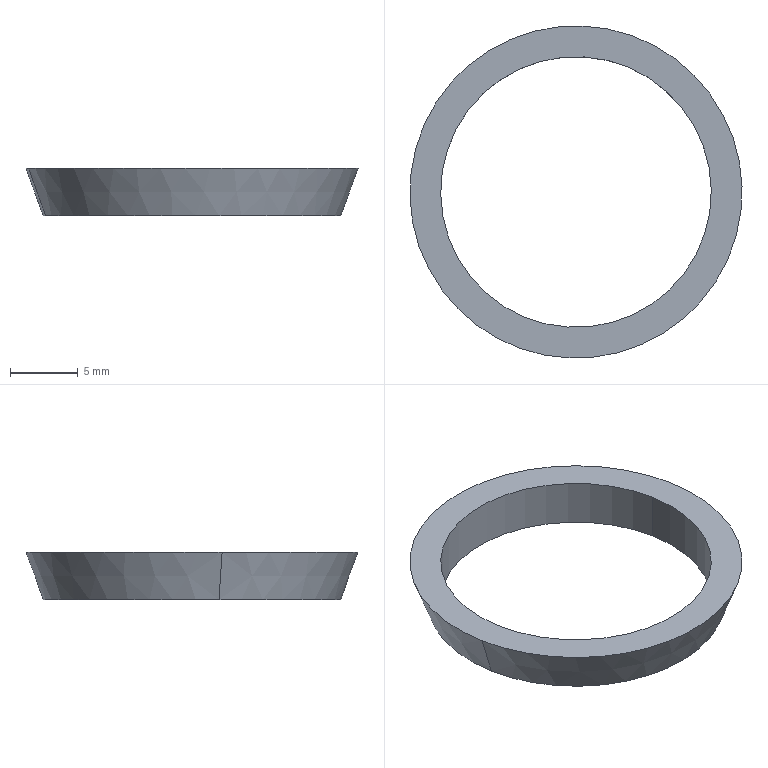Component | SolidWorks | OilSeal-1 | 1 solid | 6 faces | box 24.55 x 24.55 x 3.5 mm | volume 391 mm3 | cylinder 2 | cone 2 | plane 2 | commonest cylinder face diameters 20 x2
build123d program:
from build123d import *

# Parameters (mm, degrees)
SKETCH2_R           = 11
SKETCH2_R_2         = 10
BOSS_EXTRUDE1_DEPTH = 3.5
BOSS_EXTRUDE1_DRAFT = -20
SKETCH3_R           = 10
CUT_EXTRUDE1_DEPTH  = 15.5


with BuildPart() as part:
    # Sketch2 → Boss-Extrude1 (with draft: the straight prism first)
    with BuildSketch(Plane.XY):
        with Locations((-80.719, -28.485)):
            Circle(SKETCH2_R)
        with Locations((-80.719, -28.485)):
            Circle(SKETCH2_R_2, mode=Mode.SUBTRACT)
    extrude(amount=BOSS_EXTRUDE1_DEPTH)
    # Boss-Extrude1: the draft: its side faces are tilted about the plane it starts from
    boss_extrude1_sides = [part.faces().sort_by_distance(p)[0] for p in [
        (-91.719, -28.485, 1.75),
        (-90.719, -28.485, 1.75),
    ]]
    draft(boss_extrude1_sides, Plane.XY, BOSS_EXTRUDE1_DRAFT)

    # Sketch3 → Cut-Extrude1 (cut)
    with BuildSketch(Plane.XY.offset(3.5)):
        with Locations((-80.719, -28.485)):
            Circle(SKETCH3_R)
    extrude(amount=-CUT_EXTRUDE1_DEPTH, mode=Mode.SUBTRACT)


solid = part.part

# Placed as in the assembly
solid = solid.moved(Location((0, 0, 213.536), (0, 0, 0)))
STEP:
#1=COLOUR_RGB('',0.7922,0.8196,0.9333);
#2=FILL_AREA_STYLE_COLOUR('',#1);
#3=FILL_AREA_STYLE('',(#2));
#4=SURFACE_STYLE_FILL_AREA(#3);
#5=SURFACE_SIDE_STYLE('',(#4));
#6=SURFACE_STYLE_USAGE(.BOTH.,#5);
#7=PRESENTATION_STYLE_ASSIGNMENT((#6));
#8=CARTESIAN_POINT('',(-2.791,-1.05,8.407));
#9=VERTEX_POINT('',#8);
#10=CARTESIAN_POINT('',(-3.565,-1.193,8.407));
#11=VERTEX_POINT('',#10);
#12=CARTESIAN_POINT('',(-3.178,-1.121,8.407));
#13=DIRECTION('',(0.,0.,-1.));
#14=DIRECTION('',(-0.9835,-0.1812,0.));
#15=AXIS2_PLACEMENT_3D('',#12,#13,#14);
#16=CIRCLE('',#15,0.3937);
#17=EDGE_CURVE('',#9,#11,#16,.T.);
#18=ORIENTED_EDGE('',*,*,#17,.T.);
#19=CARTESIAN_POINT('',(-3.565,-1.193,8.545));
#20=VERTEX_POINT('',#19);
#21=CARTESIAN_POINT('',(-3.565,-1.193,7.934));
#22=DIRECTION('',(0.,0.,1.));
#23=VECTOR('',#22,39.37);
#24=LINE('',#21,#23);
#25=EDGE_CURVE('',#11,#20,#24,.T.);
#26=ORIENTED_EDGE('',*,*,#25,.T.);
#27=CARTESIAN_POINT('',(-2.791,-1.05,8.545));
#28=VERTEX_POINT('',#27);
#29=CARTESIAN_POINT('',(-3.178,-1.121,8.545));
#30=DIRECTION('',(0.,0.,1.));
#31=DIRECTION('',(0.9835,0.1812,0.));
#32=AXIS2_PLACEMENT_3D('',#29,#30,#31);
#33=CIRCLE('',#32,0.3937);
#34=EDGE_CURVE('',#20,#28,#33,.T.);
#35=ORIENTED_EDGE('',*,*,#34,.T.);
#36=CARTESIAN_POINT('',(-2.791,-1.05,7.934));
#37=DIRECTION('',(0.,0.,1.));
#38=VECTOR('',#37,39.37);
#39=LINE('',#36,#38);
#40=EDGE_CURVE('',#9,#28,#39,.T.);
#41=ORIENTED_EDGE('',*,*,#40,.F.);
#42=EDGE_LOOP('',(#18,#26,#35,#41));
#43=FACE_OUTER_BOUND('',#42,.T.);
#44=CARTESIAN_POINT('',(-3.178,-1.121,7.934));
#45=DIRECTION('',(0.,0.,1.));
#46=DIRECTION('',(0.9835,0.1812,0.));
#47=AXIS2_PLACEMENT_3D('',#44,#45,#46);
#48=CYLINDRICAL_SURFACE('',#47,0.3937);
#49=ADVANCED_FACE('',(#43),#48,.F.);
#50=CARTESIAN_POINT('',(-2.752,-1.043,8.407));
#51=VERTEX_POINT('',#50);
#52=CARTESIAN_POINT('',(-3.604,-1.2,8.407));
#53=VERTEX_POINT('',#52);
#54=CARTESIAN_POINT('',(-3.178,-1.121,8.407));
#55=DIRECTION('',(0.,0.,1.));
#56=DIRECTION('',(0.9835,0.1812,0.));
#57=AXIS2_PLACEMENT_3D('',#54,#55,#56);
#58=CIRCLE('',#57,0.4331);
#59=EDGE_CURVE('',#51,#53,#58,.T.);
#60=ORIENTED_EDGE('',*,*,#59,.T.);
#61=CARTESIAN_POINT('',(-3.653,-1.209,8.545));
#62=VERTEX_POINT('',#61);
#63=CARTESIAN_POINT('',(-3.604,-1.2,8.407));
#64=DIRECTION('',(-0.3364,-0.06196,0.9397));
#65=VECTOR('',#64,39.37);
#66=LINE('',#63,#65);
#67=EDGE_CURVE('',#53,#62,#66,.T.);
#68=ORIENTED_EDGE('',*,*,#67,.T.);
#69=CARTESIAN_POINT('',(-2.703,-1.034,8.545));
#70=VERTEX_POINT('',#69);
#71=CARTESIAN_POINT('',(-3.178,-1.121,8.545));
#72=DIRECTION('',(0.,0.,1.));
#73=DIRECTION('',(0.9835,0.1812,0.));
#74=AXIS2_PLACEMENT_3D('',#71,#72,#73);
#75=CIRCLE('',#74,0.4832);
#76=EDGE_CURVE('',#70,#62,#75,.T.);
#77=ORIENTED_EDGE('',*,*,#76,.F.);
#78=CARTESIAN_POINT('',(-2.752,-1.043,8.407));
#79=DIRECTION('',(0.3364,0.06196,0.9397));
#80=VECTOR('',#79,39.37);
#81=LINE('',#78,#80);
#82=EDGE_CURVE('',#51,#70,#81,.T.);
#83=ORIENTED_EDGE('',*,*,#82,.F.);
#84=EDGE_LOOP('',(#60,#68,#77,#83));
#85=FACE_OUTER_BOUND('',#84,.T.);
#86=CARTESIAN_POINT('',(-3.178,-1.121,8.407));
#87=DIRECTION('',(0.,0.,1.));
#88=DIRECTION('',(0.9835,0.1812,0.));
#89=AXIS2_PLACEMENT_3D('',#86,#87,#88);
#90=CONICAL_SURFACE('',#89,0.4331,0.3491);
#91=ADVANCED_FACE('',(#85),#90,.T.);
#92=CARTESIAN_POINT('',(-3.178,-1.121,8.545));
#93=DIRECTION('',(0.,0.,1.));
#94=DIRECTION('',(0.9835,0.1812,0.));
#95=AXIS2_PLACEMENT_3D('',#92,#93,#94);
#96=CIRCLE('',#95,0.3937);
#97=EDGE_CURVE('',#28,#20,#96,.T.);
#98=ORIENTED_EDGE('',*,*,#97,.F.);
#99=ORIENTED_EDGE('',*,*,#34,.F.);
#100=EDGE_LOOP('',(#98,#99));
#101=FACE_BOUND('',#100,.T.);
#102=ORIENTED_EDGE('',*,*,#76,.T.);
#103=CARTESIAN_POINT('',(-3.178,-1.121,8.545));
#104=DIRECTION('',(0.,0.,1.));
#105=DIRECTION('',(0.9835,0.1812,0.));
#106=AXIS2_PLACEMENT_3D('',#103,#104,#105);
#107=CIRCLE('',#106,0.4832);
#108=EDGE_CURVE('',#62,#70,#107,.T.);
#109=ORIENTED_EDGE('',*,*,#108,.T.);
#110=EDGE_LOOP('',(#102,#109));
#111=FACE_OUTER_BOUND('',#110,.T.);
#112=CARTESIAN_POINT('',(-3.178,-1.121,8.545));
#113=DIRECTION('',(0.,0.,1.));
#114=DIRECTION('',(0.9835,0.1812,0.));
#115=AXIS2_PLACEMENT_3D('',#112,#113,#114);
#116=PLANE('',#115);
#117=ADVANCED_FACE('',(#101,#111),#116,.T.);
#118=ORIENTED_EDGE('',*,*,#59,.F.);
#119=CARTESIAN_POINT('',(-3.178,-1.121,8.407));
#120=DIRECTION('',(0.,0.,1.));
#121=DIRECTION('',(0.9835,0.1812,0.));
#122=AXIS2_PLACEMENT_3D('',#119,#120,#121);
#123=CIRCLE('',#122,0.4331);
#124=EDGE_CURVE('',#53,#51,#123,.T.);
#125=ORIENTED_EDGE('',*,*,#124,.F.);
#126=EDGE_LOOP('',(#118,#125));
#127=FACE_OUTER_BOUND('',#126,.T.);
#128=ORIENTED_EDGE('',*,*,#17,.F.);
#129=CARTESIAN_POINT('',(-3.178,-1.121,8.407));
#130=DIRECTION('',(0.,0.,-1.));
#131=DIRECTION('',(-0.9835,-0.1812,0.));
#132=AXIS2_PLACEMENT_3D('',#129,#130,#131);
#133=CIRCLE('',#132,0.3937);
#134=EDGE_CURVE('',#11,#9,#133,.T.);
#135=ORIENTED_EDGE('',*,*,#134,.F.);
#136=EDGE_LOOP('',(#128,#135));
#137=FACE_BOUND('',#136,.T.);
#138=CARTESIAN_POINT('',(-3.178,-1.121,8.407));
#139=DIRECTION('',(0.,0.,1.));
#140=DIRECTION('',(0.9835,0.1812,0.));
#141=AXIS2_PLACEMENT_3D('',#138,#139,#140);
#142=PLANE('',#141);
#143=ADVANCED_FACE('',(#127,#137),#142,.F.);
#144=ORIENTED_EDGE('',*,*,#67,.F.);
#145=ORIENTED_EDGE('',*,*,#124,.T.);
#146=ORIENTED_EDGE('',*,*,#82,.T.);
#147=ORIENTED_EDGE('',*,*,#108,.F.);
#148=EDGE_LOOP('',(#144,#145,#146,#147));
#149=FACE_OUTER_BOUND('',#148,.T.);
#150=CARTESIAN_POINT('',(-3.178,-1.121,8.407));
#151=DIRECTION('',(0.,0.,1.));
#152=DIRECTION('',(0.9835,0.1812,0.));
#153=AXIS2_PLACEMENT_3D('',#150,#151,#152);
#154=CONICAL_SURFACE('',#153,0.4331,0.3491);
#155=ADVANCED_FACE('',(#149),#154,.T.);
#156=ORIENTED_EDGE('',*,*,#25,.F.);
#157=ORIENTED_EDGE('',*,*,#134,.T.);
#158=ORIENTED_EDGE('',*,*,#40,.T.);
#159=ORIENTED_EDGE('',*,*,#97,.T.);
#160=EDGE_LOOP('',(#156,#157,#158,#159));
#161=FACE_OUTER_BOUND('',#160,.T.);
#162=CARTESIAN_POINT('',(-3.178,-1.121,7.934));
#163=DIRECTION('',(0.,0.,1.));
#164=DIRECTION('',(0.9835,0.1812,0.));
#165=AXIS2_PLACEMENT_3D('',#162,#163,#164);
#166=CYLINDRICAL_SURFACE('',#165,0.3937);
#167=ADVANCED_FACE('',(#161),#166,.F.);
#168=CLOSED_SHELL('',(#49,#91,#117,#143,#155,#167));
#169=MANIFOLD_SOLID_BREP('',#168);
#170=STYLED_ITEM('',(#7),#169);
#171=(LENGTH_UNIT()NAMED_UNIT(*)SI_UNIT($,.METRE.));
#172=LENGTH_MEASURE_WITH_UNIT(LENGTH_MEASURE(0.0254),#171);
#173=DIMENSIONAL_EXPONENTS(1.,0.,0.,0.,0.,0.,0.);
#174=(CONVERSION_BASED_UNIT('',#172)LENGTH_UNIT()NAMED_UNIT(#173));
#175=UNCERTAINTY_MEASURE_WITH_UNIT(LENGTH_MEASURE(0.00001),#174,'','');
#176=(NAMED_UNIT(*)PLANE_ANGLE_UNIT()SI_UNIT($,.RADIAN.));
#177=(NAMED_UNIT(*)SI_UNIT($,.STERADIAN.)SOLID_ANGLE_UNIT());
#178=(GEOMETRIC_REPRESENTATION_CONTEXT(3)GLOBAL_UNCERTAINTY_ASSIGNED_CONTEXT((#175))GLOBAL_UNIT_ASSIGNED_CONTEXT((#174,#176,#177))REPRESENTATION_CONTEXT('',''));
#179=MECHANICAL_DESIGN_GEOMETRIC_PRESENTATION_REPRESENTATION('',(#170),#178);
#180=PRESENTATION_LAYER_ASSIGNMENT('','',(#170));
#181=CARTESIAN_POINT('',(0.,0.,0.));
#182=DIRECTION('',(0.,0.,1.));
#183=DIRECTION('',(1.,0.,0.));
#184=AXIS2_PLACEMENT_3D('',#181,#182,#183);
#185=(LENGTH_UNIT()NAMED_UNIT(*)SI_UNIT($,.METRE.));
#186=LENGTH_MEASURE_WITH_UNIT(LENGTH_MEASURE(0.0254),#185);
#187=DIMENSIONAL_EXPONENTS(1.,0.,0.,0.,0.,0.,0.);
#188=(CONVERSION_BASED_UNIT('',#186)LENGTH_UNIT()NAMED_UNIT(#187));
#189=UNCERTAINTY_MEASURE_WITH_UNIT(LENGTH_MEASURE(0.00001),#188,'','');
#190=(NAMED_UNIT(*)PLANE_ANGLE_UNIT()SI_UNIT($,.RADIAN.));
#191=(NAMED_UNIT(*)SI_UNIT($,.STERADIAN.)SOLID_ANGLE_UNIT());
#192=(GEOMETRIC_REPRESENTATION_CONTEXT(3)GLOBAL_UNCERTAINTY_ASSIGNED_CONTEXT((#189))GLOBAL_UNIT_ASSIGNED_CONTEXT((#188,#190,#191))REPRESENTATION_CONTEXT('',''));
#193=ADVANCED_BREP_SHAPE_REPRESENTATION('',(#169,#184),#192);